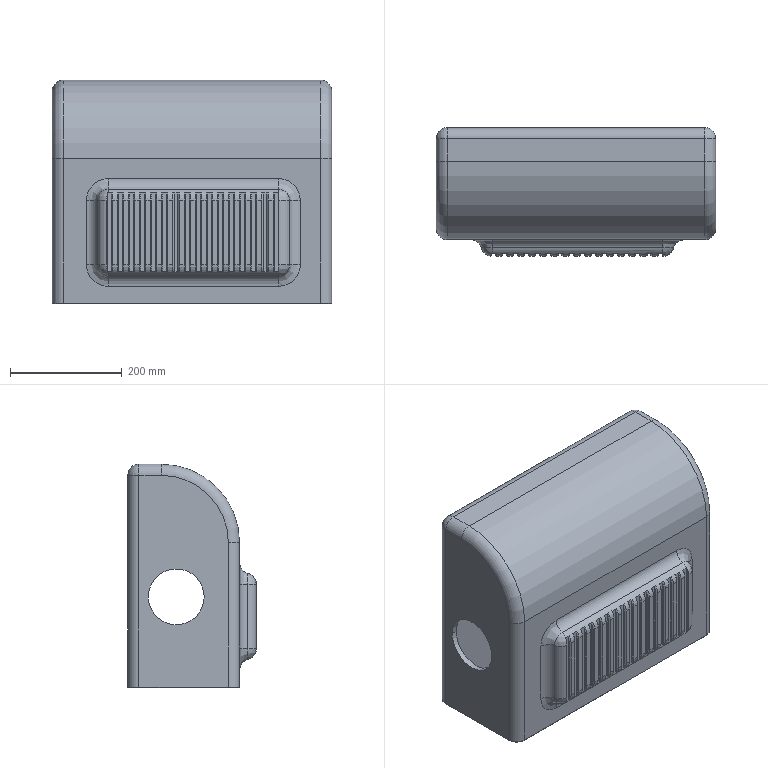Component | SolidWorks | UpperHousing-1 | 1 solid | 243 faces | volume 5882186 mm3 | plane 115 | cone 68 | cylinder 36 | spline 16 | torus 4 | sphere 4 | commonest cylinder face diameters 40 x15 20 x11 100 x4 60 x4 259.779 x1 279.779 x1